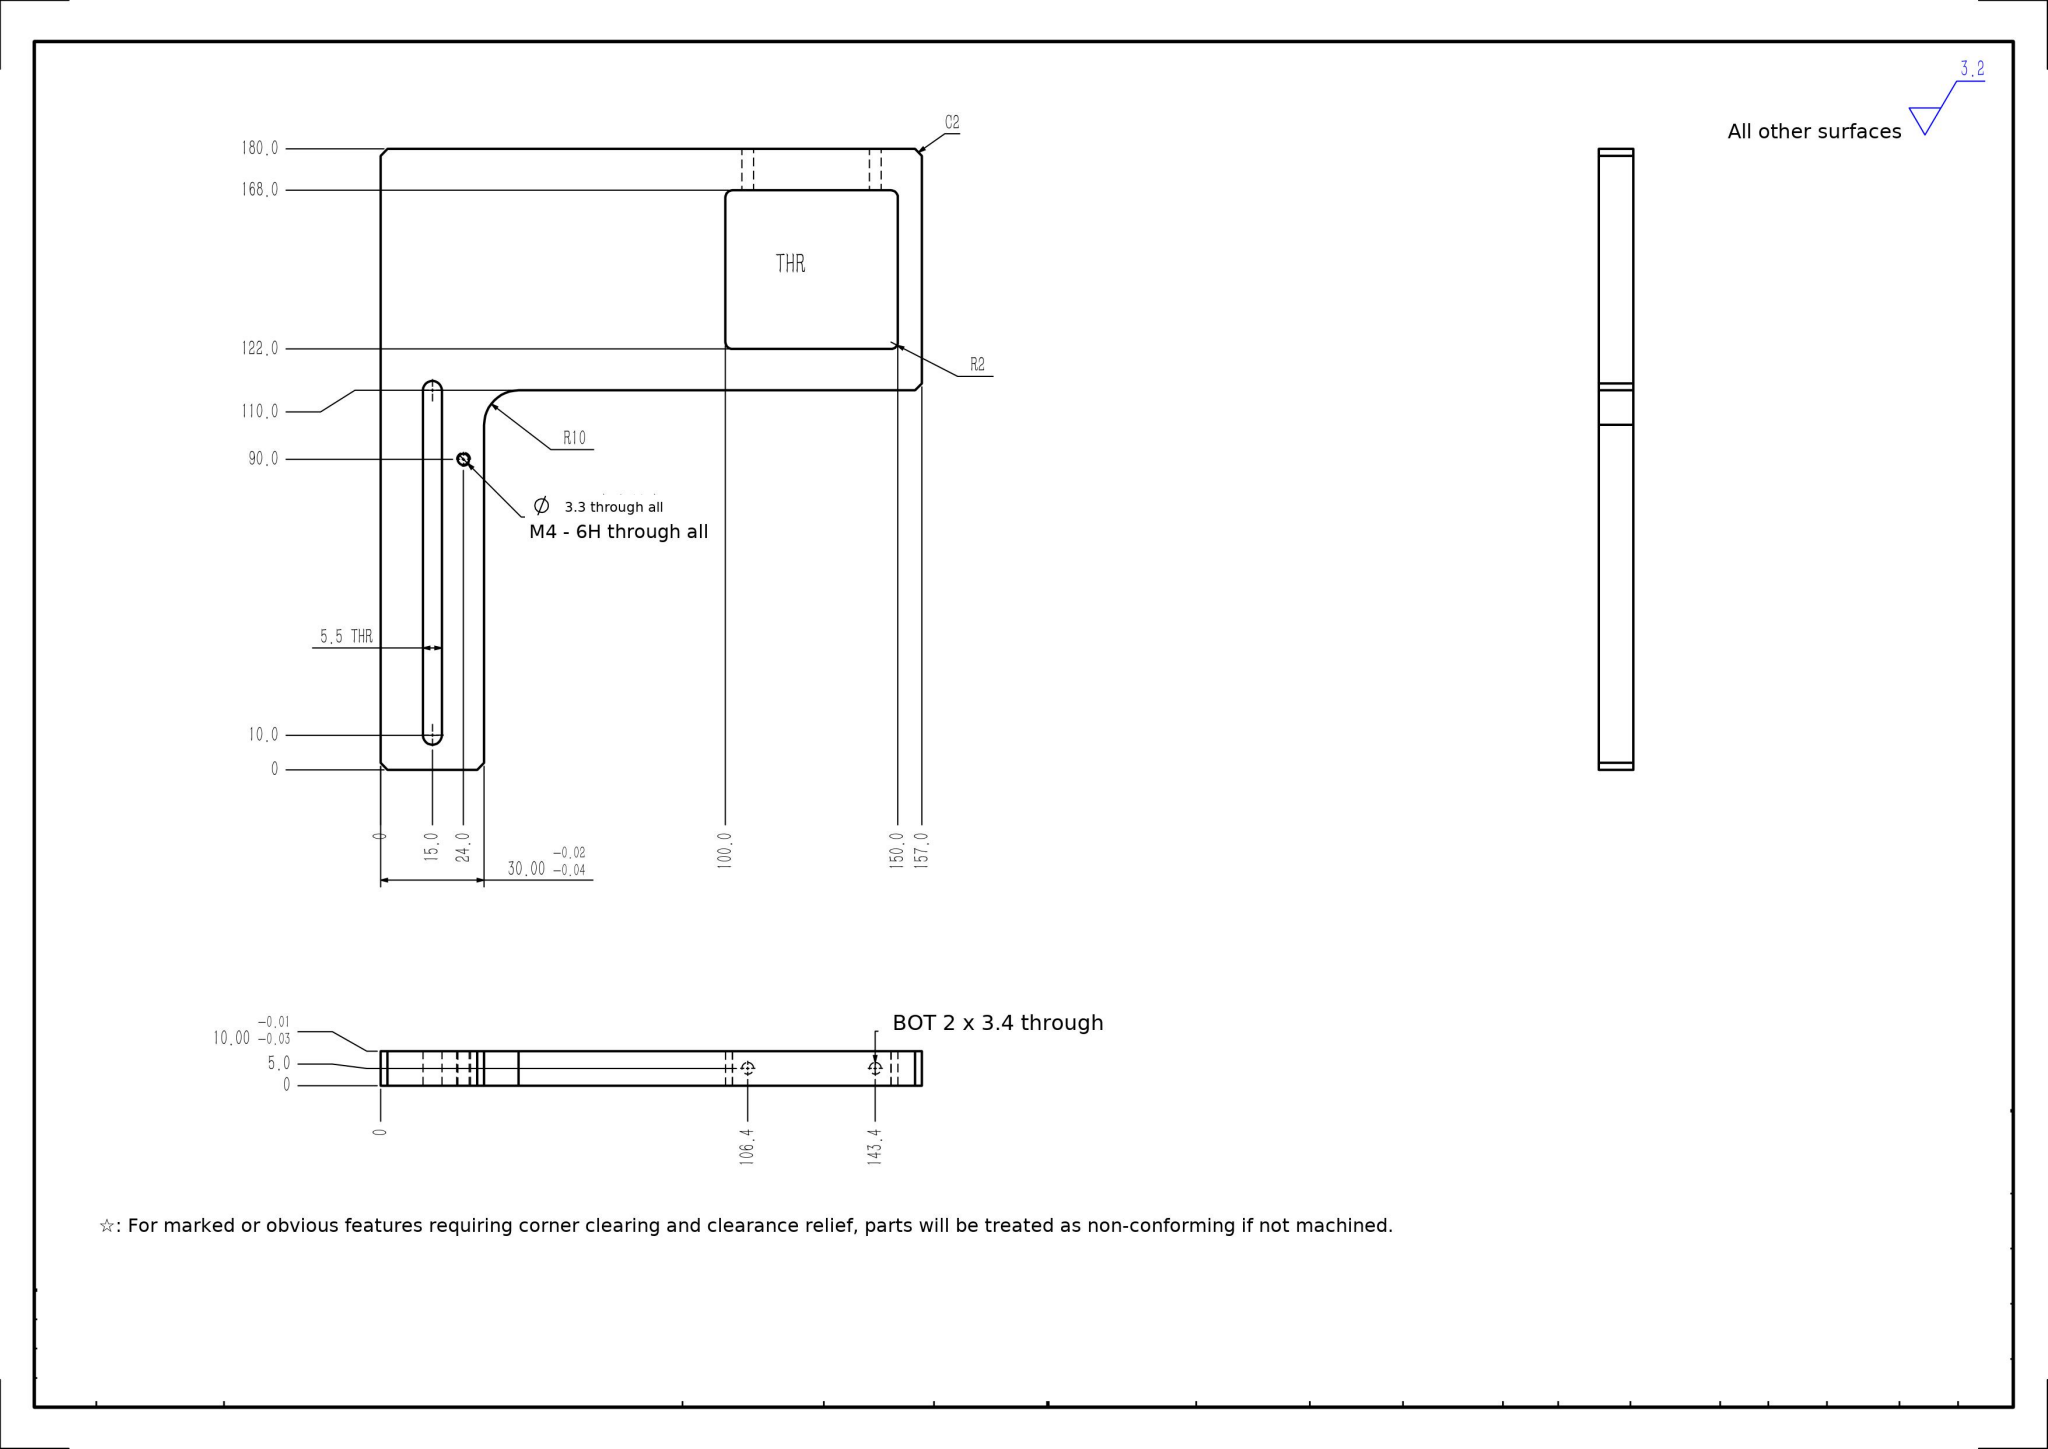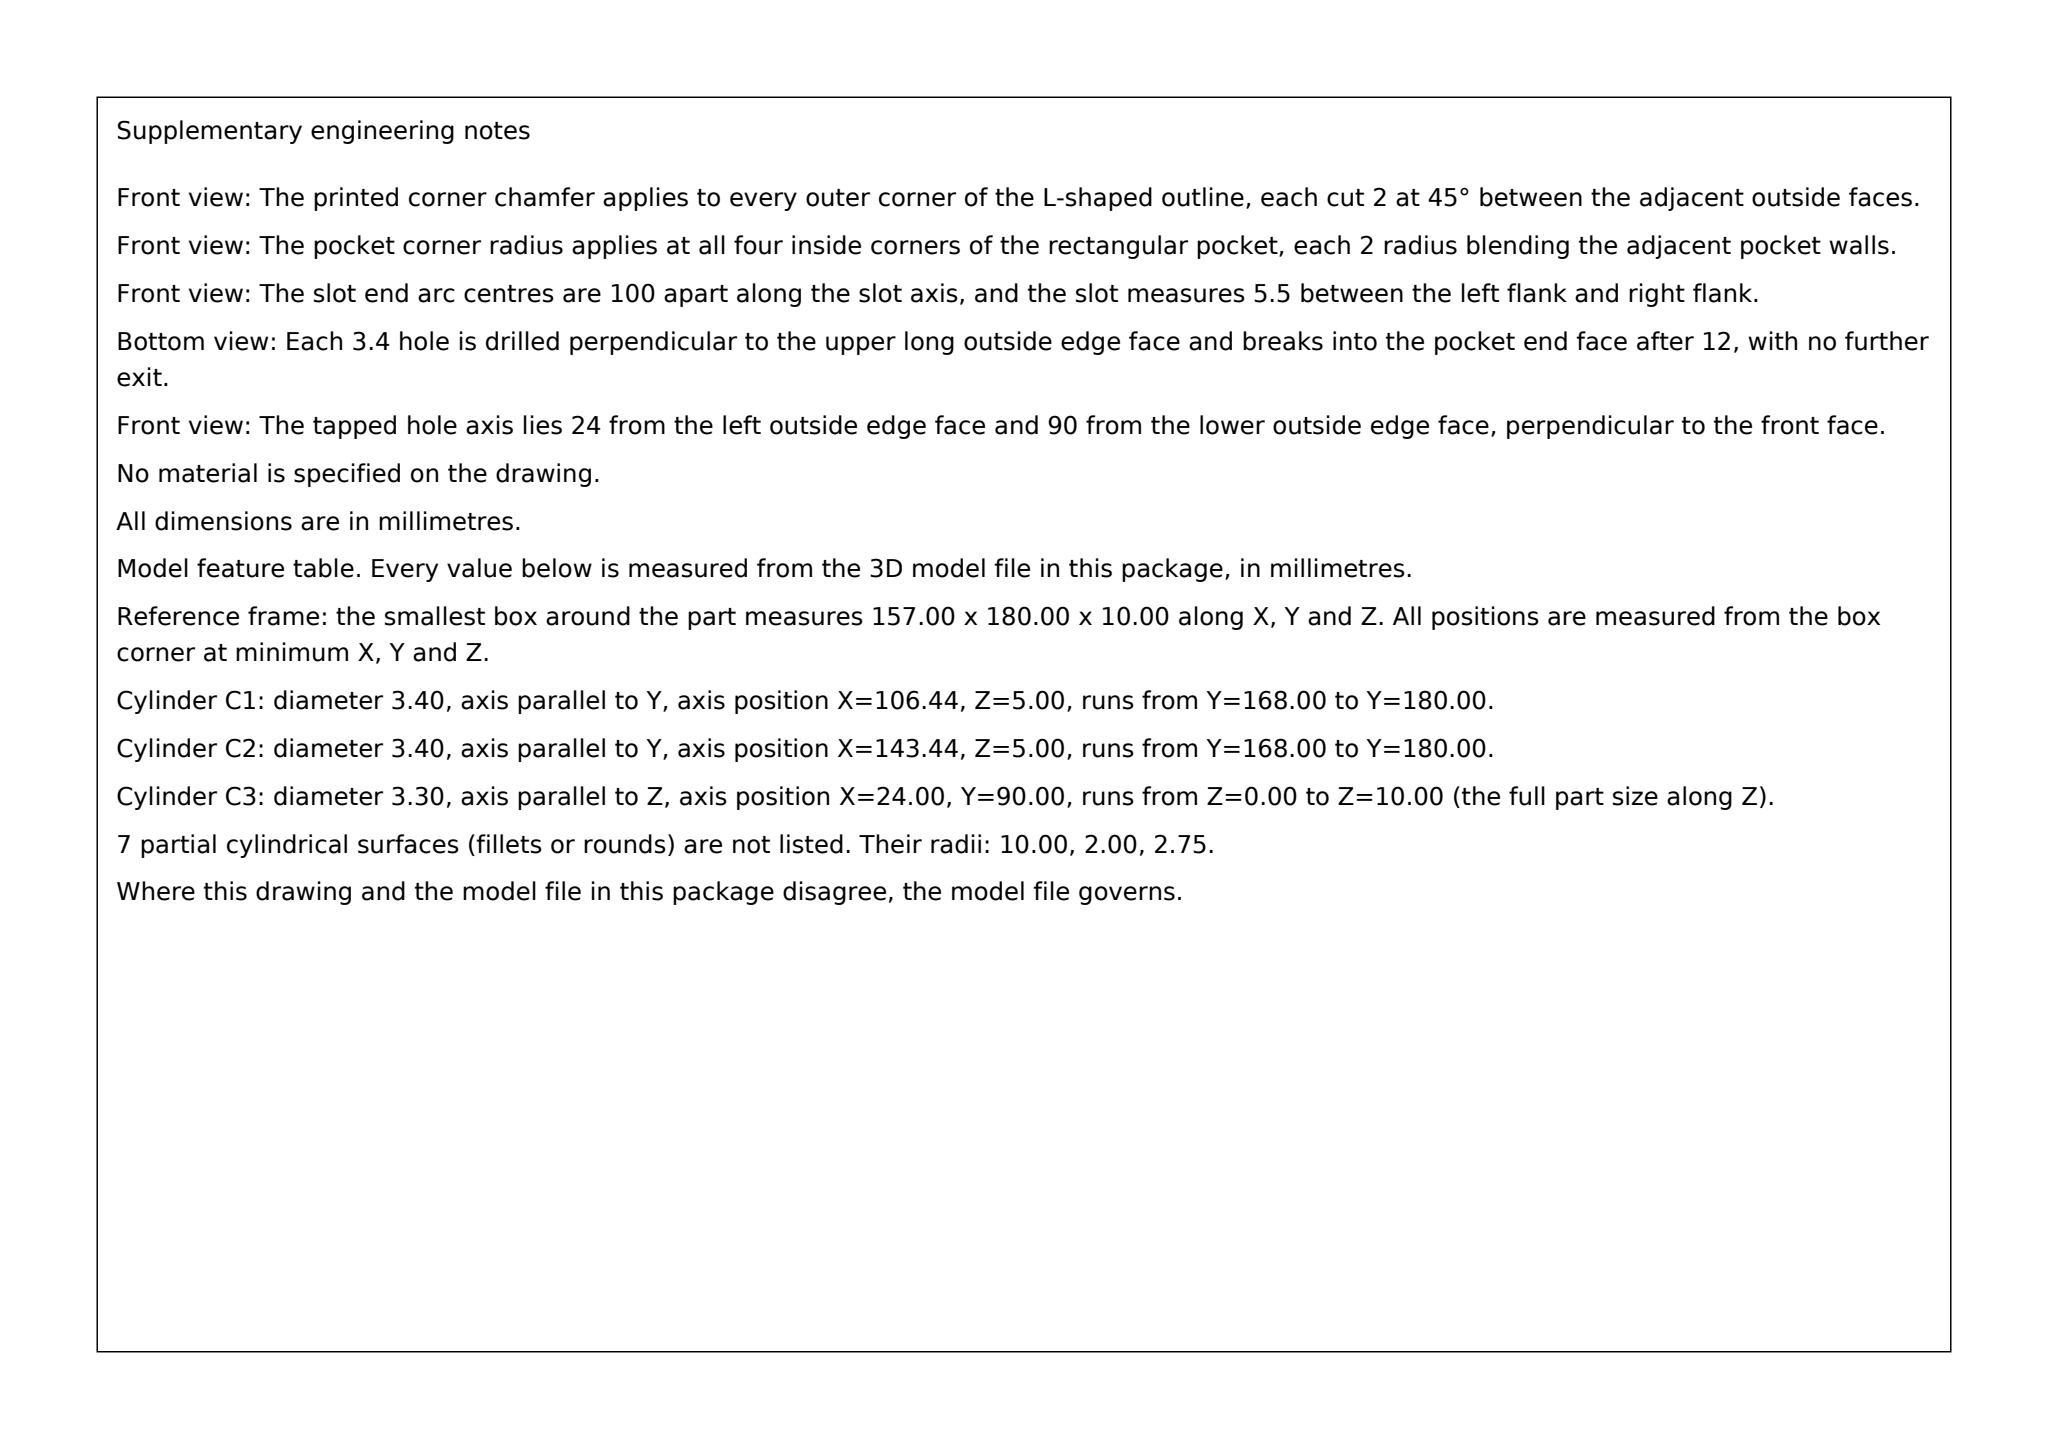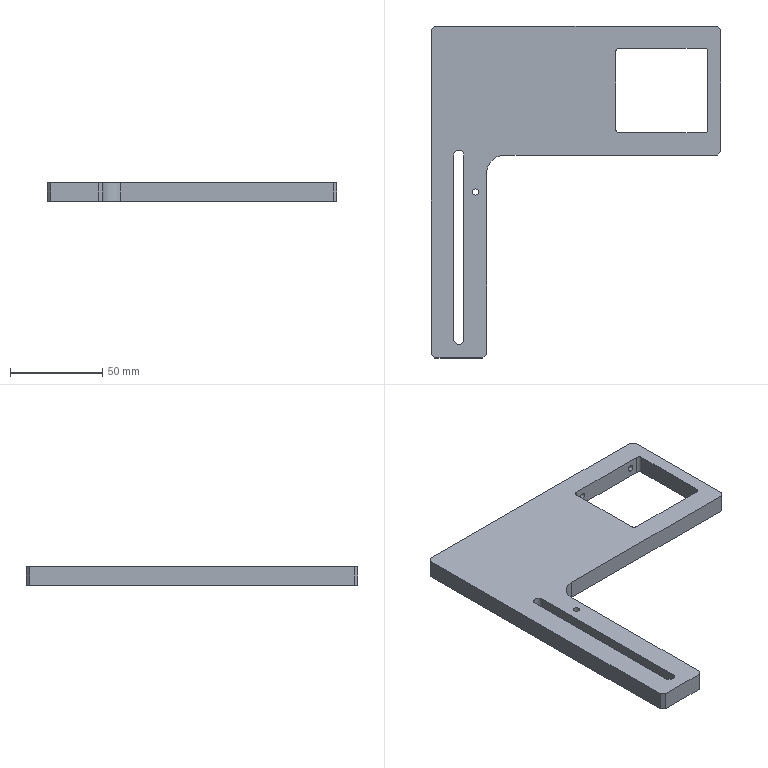Part | SolidWorks | mm | 1 solid | 32 faces | box 157 x 180 x 10 mm | volume 114008 mm3 | plane 19 | cylinder 13 | commonest cylinder face diameters 3.4 x4 4 x4 3.3 x2 5.5 x2 20 x1
Drawing notes:
BOT 2 X Ø3.4 DP 12 (NOT THRU) | from the solid: cylinders dia 3.4, axis y, pos (106.44,z5.0) & (143.44,z5.0), length 12 from y=0 BOT face
M4-6H AT X24.0 Y90.0: TAP THRU 10 THK, Ø3.3 DRILL THRU | from the solid: cylinder dia 3.3, axis z, pos [24.0, 90.0], length 10.0 = full 10.0 plate thickness (z planes 0.0 and 10.0)